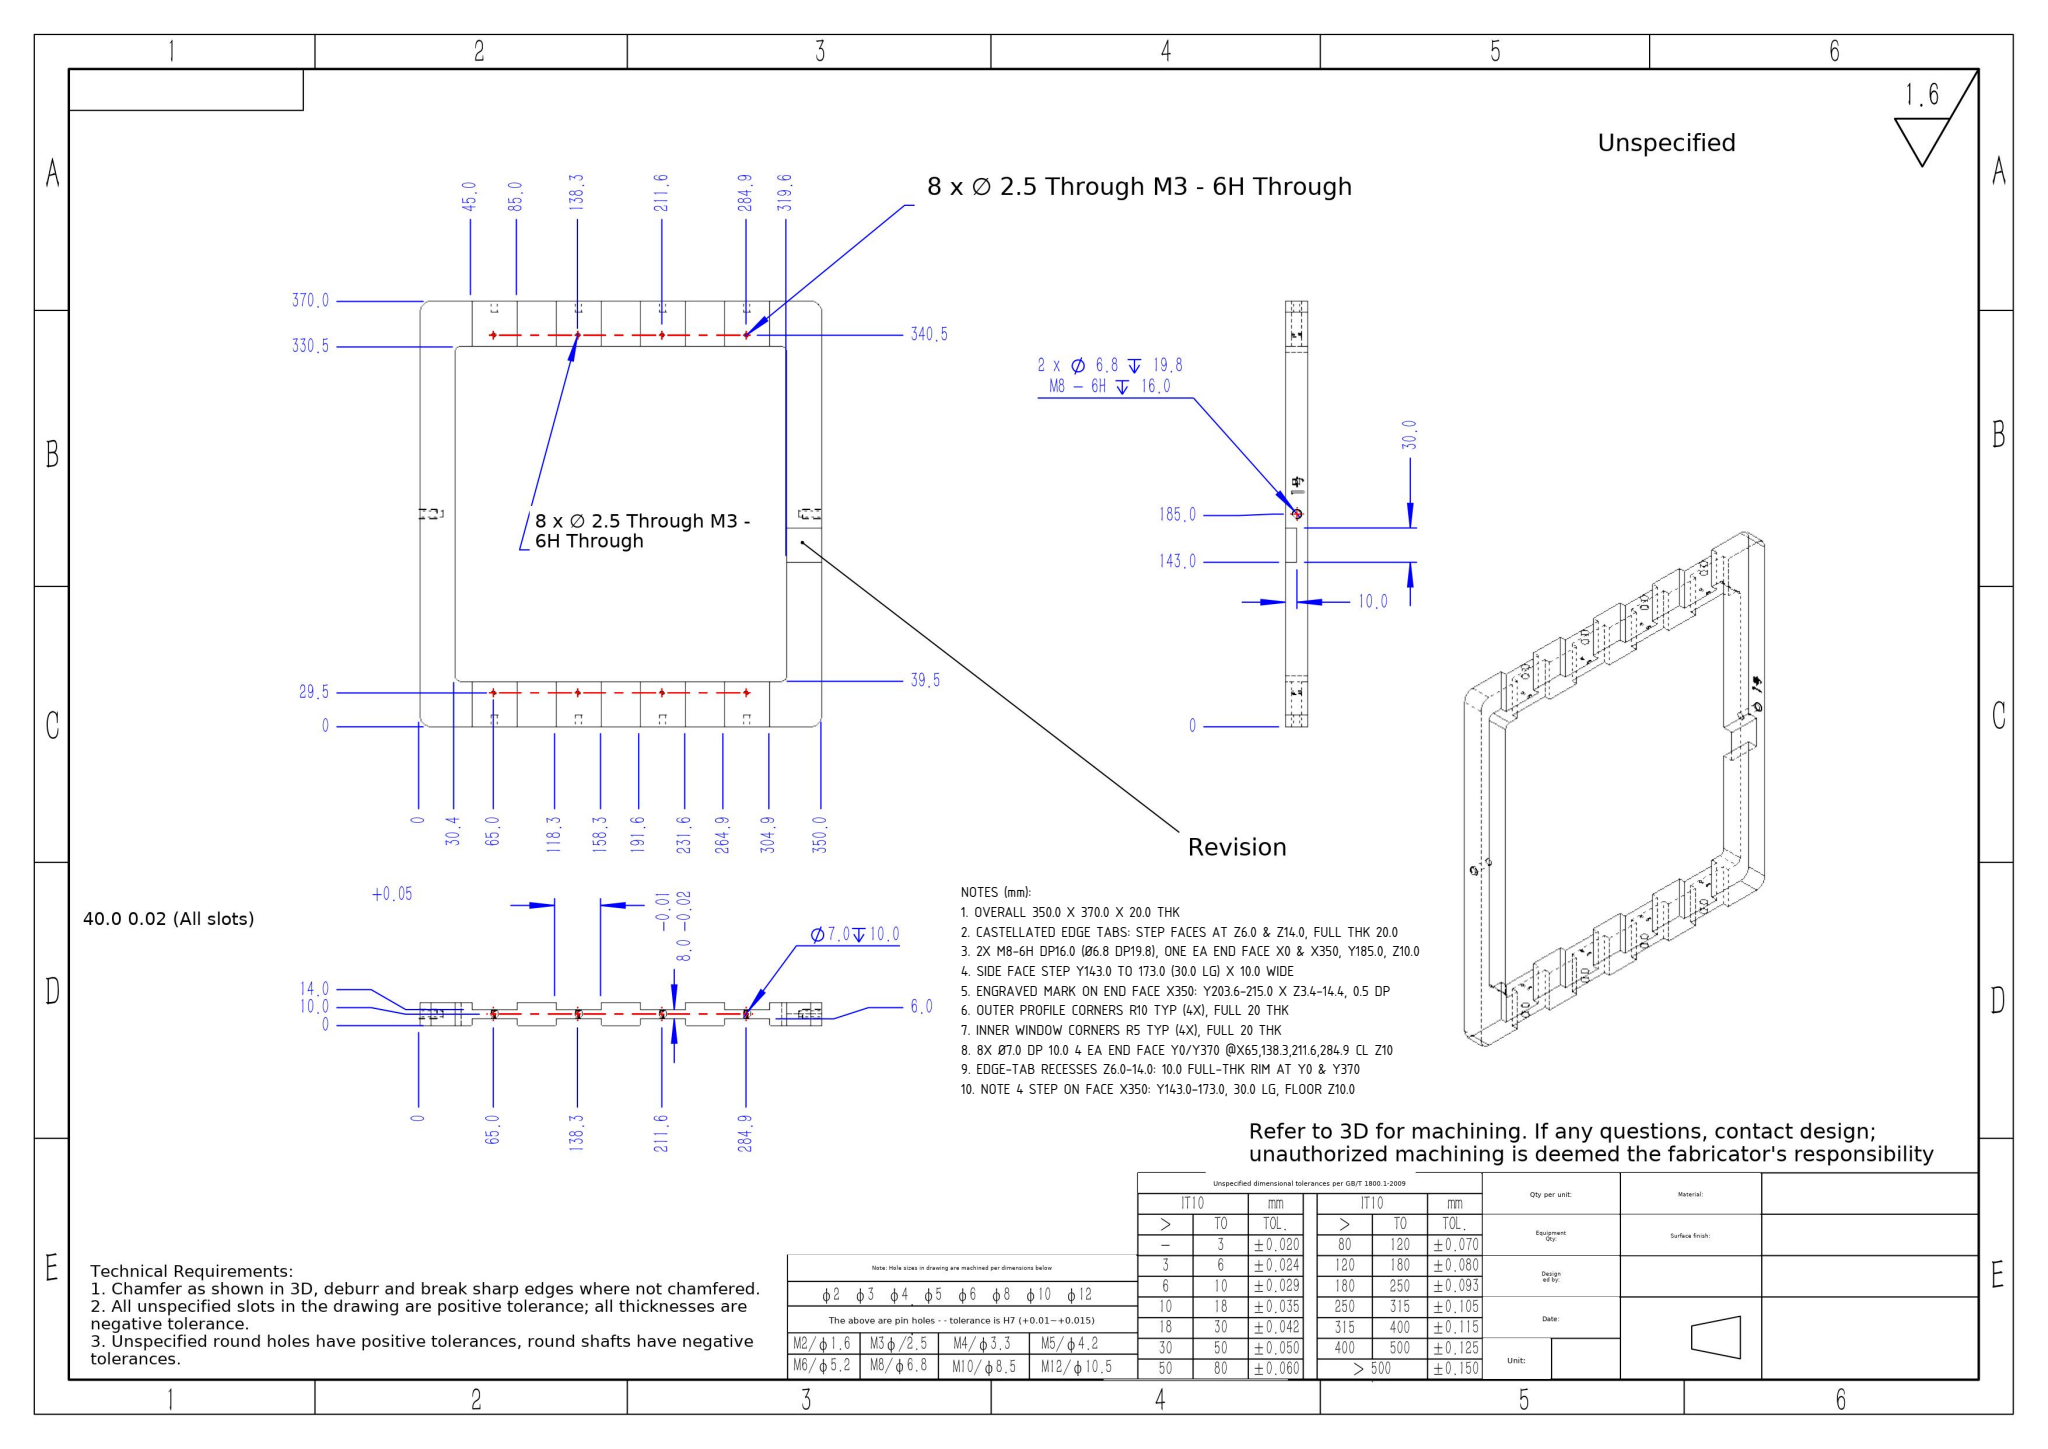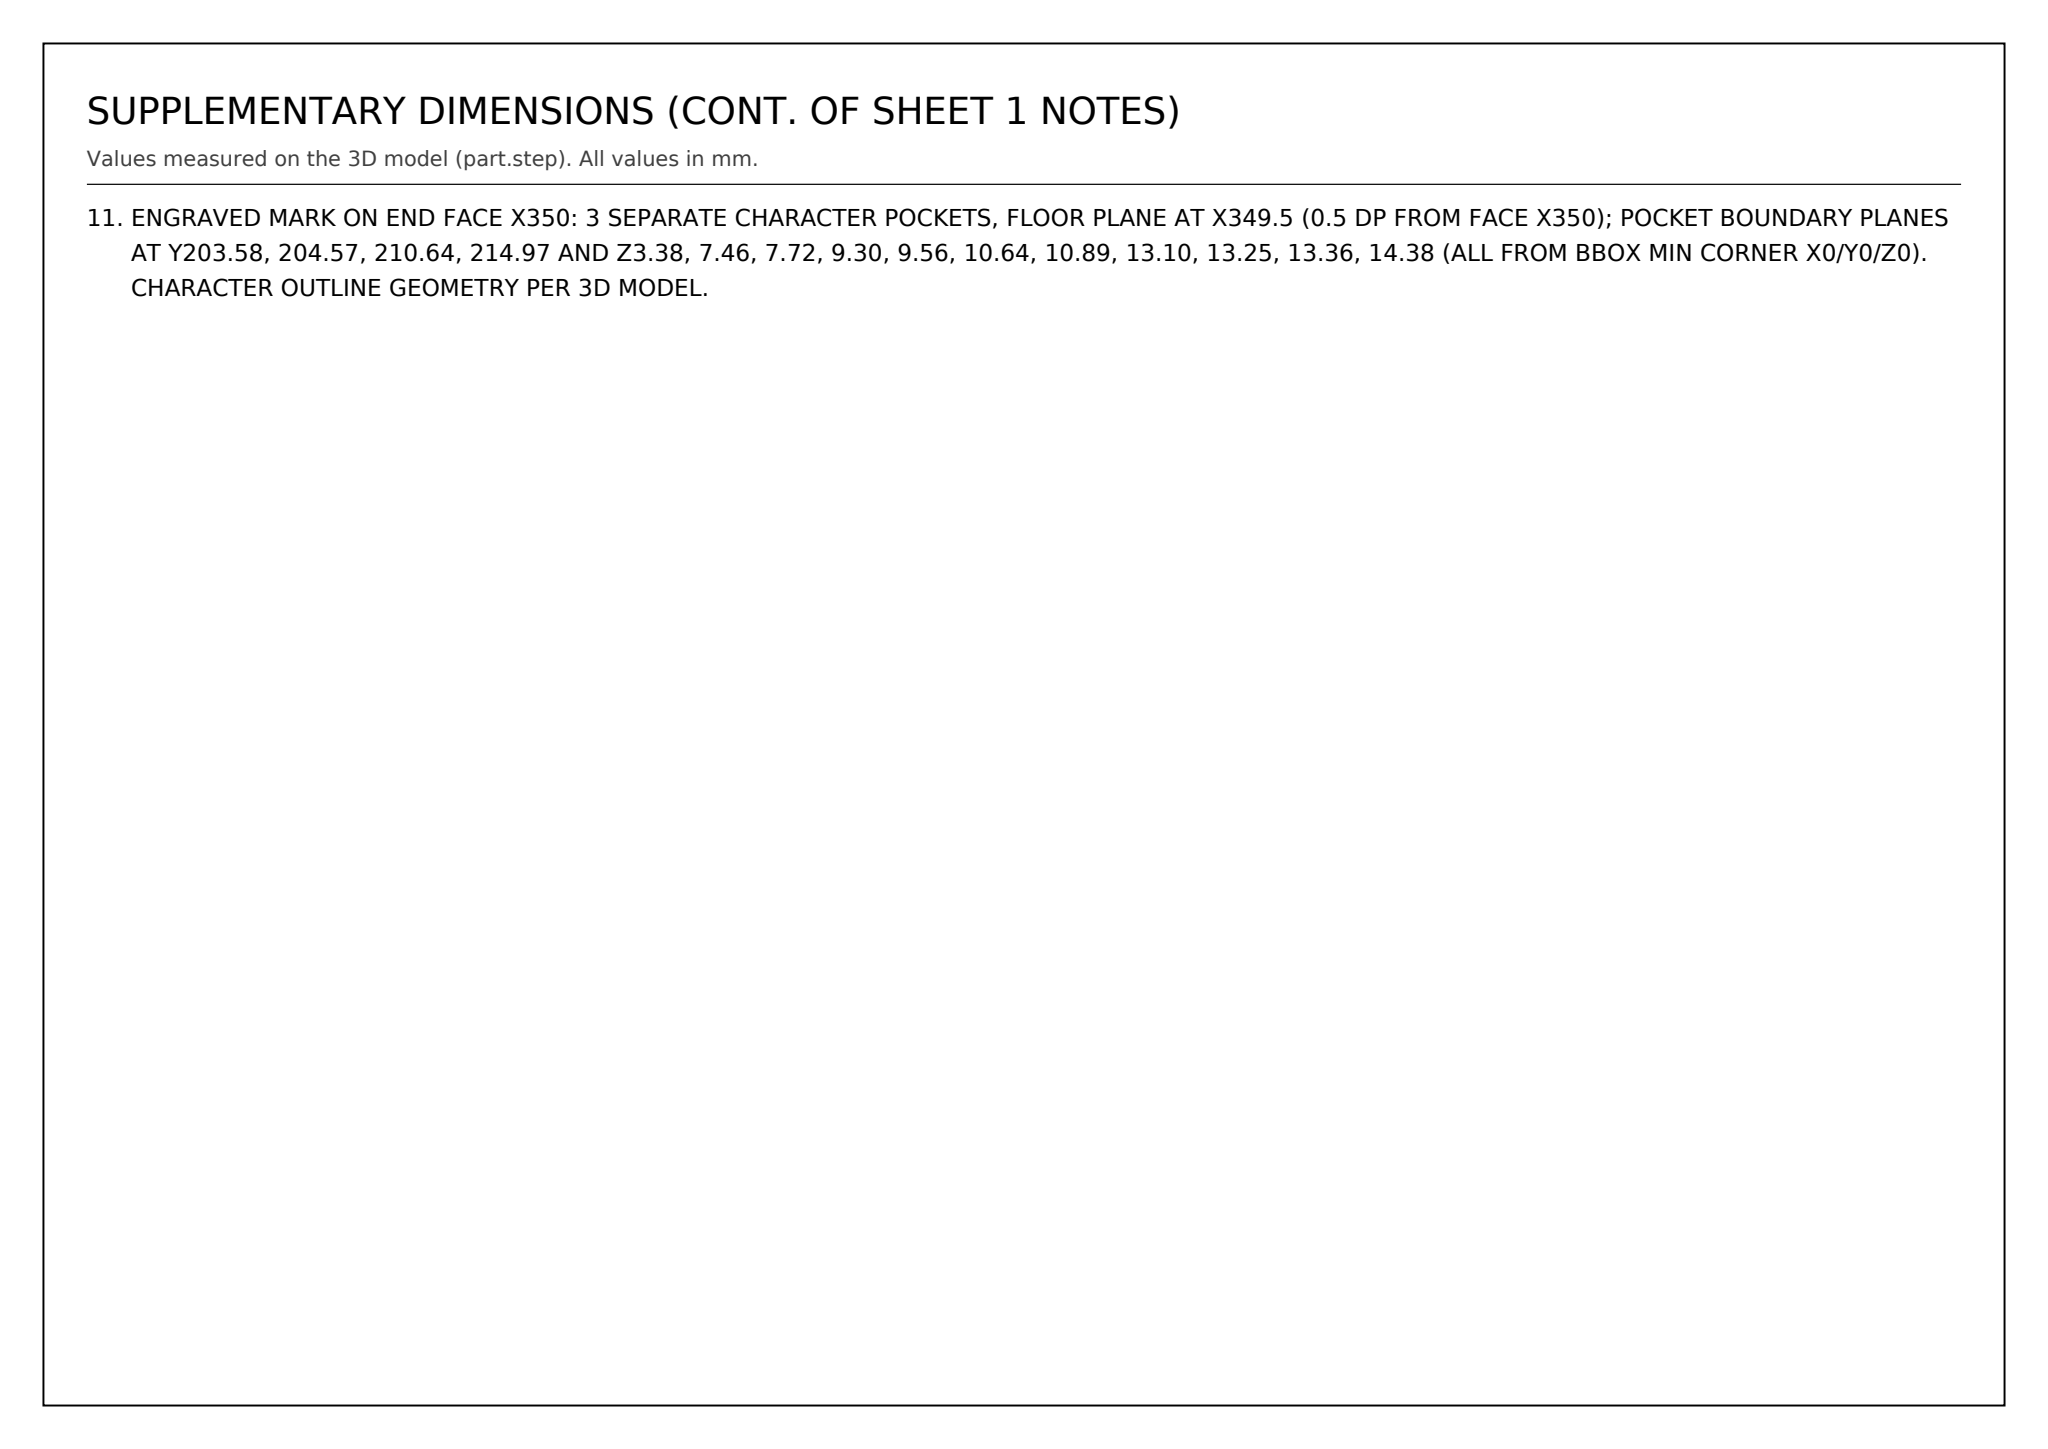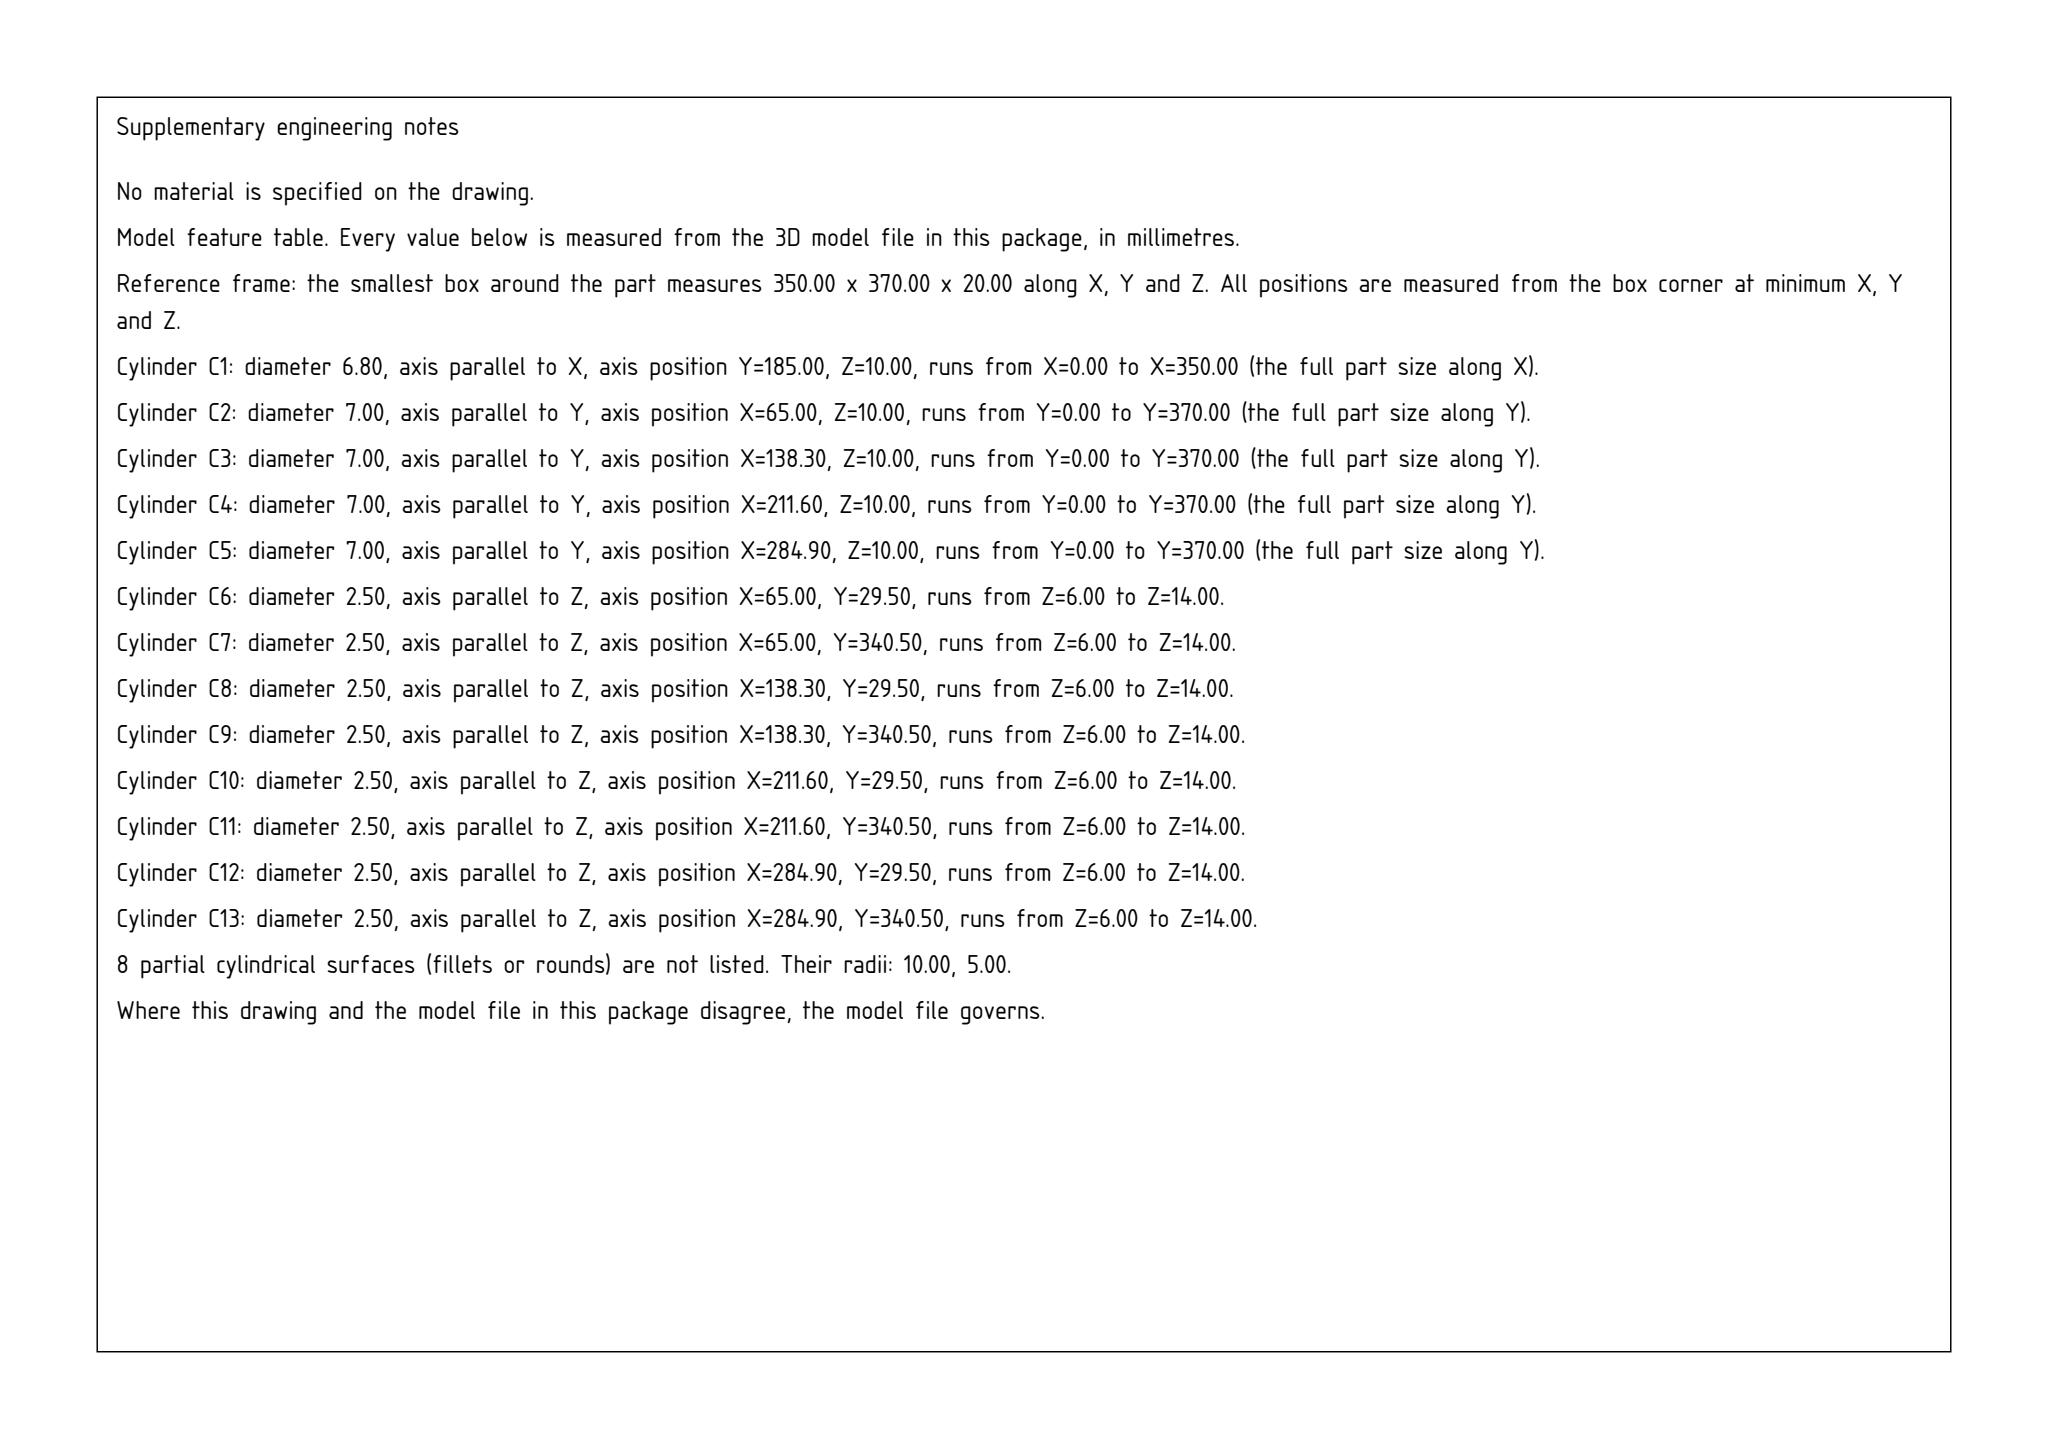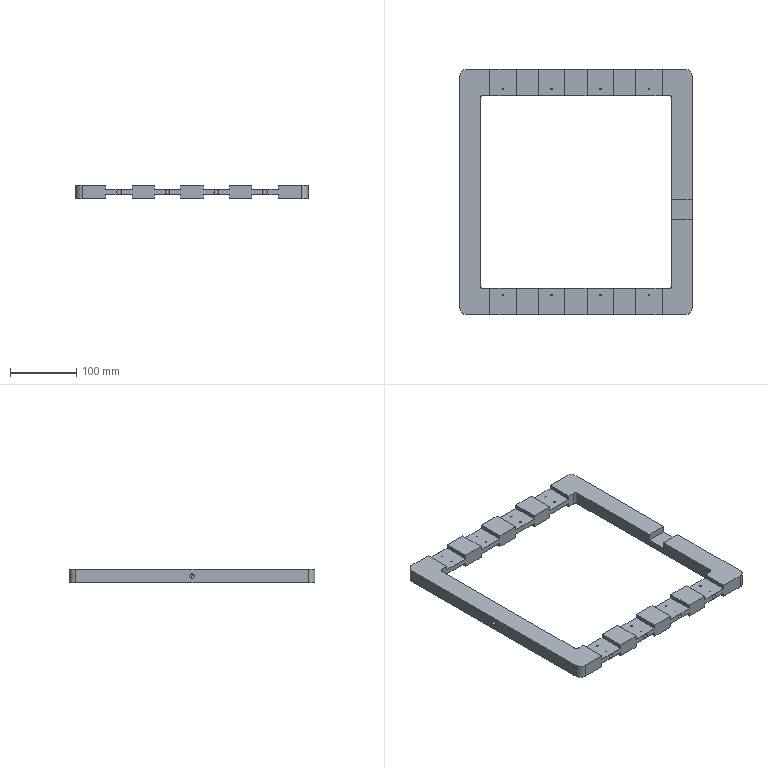Part | SolidWorks | mm | 1 solid | 179 faces | box 350 x 370 x 20 mm | volume 739874 mm3 | plane 124 | cylinder 44 | spline 7 | cone 4 | commonest cylinder face diameters 2.5 x16 7 x16 6.8 x4 20 x4 10 x4
Drawing notes:
OVERALL 350.0 X 370.0 X 20.0 THK | from the solid: bbox_xyz 350.0 x 370.0 x 20.0
CASTELLATED EDGE TABS: STEP FACES AT Z6.0 & Z14.0, FULL THK 20.0 | from the solid: z planes 0, 6.0, 14.0, 20.0, 8 faces each on tab edges
2X M8-6H DP16.0 (Ø6.8 DP19.8), ONE EA END FACE X0 & X350, Y185.0, Z10.0 | from the solid: Ø6.8 axis x at [-,185.0,10.0] L19.8, both x=0 and x=350 faces
SIDE FACE STEP Y143.0 TO 173.0 (30.0 LG) X 10.0 WIDE | from the solid: y planes 143.0 & 173.0 (delta 30.0); 10.0 width dim in right view
ENGRAVED MARK ON END FACE X350: Y203.6-215.0 X Z3.4-14.4, 0.5 DP | from the solid: x planes 349.5 & 350.0 (0.5 deep); y 203.58-214.97; z 3.38-14.38
OUTER PROFILE CORNERS R10 TYP (4X), FULL 20 THK | from the solid: Ø20 z-axis cylinders at (10,10),(10,360),(340,10),(340,360), len 20 = R10 at the 4 bbox corners of 350x370x20
INNER WINDOW CORNERS R5 TYP (4X), FULL 20 THK | from the solid: Ø10 z-axis cylinders at (35.4,44.5),(35.4,325.5),(314.6,44.5),(314.6,325.5), len 20 = R5 at pocket corners
8X Ø7.0 DP 10.0 4 EA END FACE Y0/Y370 @X65,138.3,211.6,284.9 CL Z10 | from the solid: Ø7.0 y-axis holes, depth 10, at X=65/138.3/211.6/284.9, Z=10, one from each of Y0 and Y370 faces (8 total)
EDGE-TAB RECESSES Z6.0-14.0: 10.0 FULL-THK RIM AT Y0 & Y370 | from the solid: y-planes 10.0 (x4) and 360.0 (x4) bound recess regions between z=6.0 and z=14.0; outer faces y=0.0 and y=370.0, bbox Y370.0
NOTE 4 STEP ON FACE X350: Y143.0-173.0, 30.0 LG, FLOOR Z10.0 | from the solid: y-planes 143.0 & 173.0 (30.0 apart), single z-plane 10.0 = step floor; x=350.0 face occurs 2x (split by step) vs x=0.0 face 1x
ENGRAVED MARK ON END FACE X350: 3 SEPARATE CHARACTER POCKETS, FLOOR PLANE AT X349.5 (0.5 DP FROM FACE X350); POCKET BOUNDARY PLANES AT Y203.58, 204.57, 210.64, 214.97 AND Z3.38, 7.46, 7.72, 9.30, 9.56, 10.64, 10.89, 13.10, 13.25, 13.36, 14.38 (ALL FROM BBOX MIN CORNER X0/Y0/Z0). CHARACTER OUTLINE GEOMETRY PER 3D MODEL. | from the solid: axis_planes[x,349.5]:3 (engraved floor, 0.5 below x=350 face); axis_planes y=203.58, 204.57, 210.64, 214.97; axis_planes z=3.38, 7.46, 7.72, 9.30, 9.56, 10.64, 10.89, 13.10, 13.25, 13.36, 14.38
build123d program:
from build123d import *

# Parameters (mm, degrees)
SKETCH1_W                 = 350
SKETCH1_H                 = 370
BOSS_EXTRUDE1_DEPTH       = 10
FILLET1_R                 = 10
SKETCH2_W                 = 289.2
SKETCH2_H                 = 291
CUT_EXTRUDE1_DEPTH        = 174
CUT_EXTRUDE2_DEPTH        = 0.5
SKETCH4_W                 = 2.202
SKETCH4_H                 = 4.327
CUT_EXTRUDE3_DEPTH        = 0.5
SKETCH5_W                 = 40
SKETCH5_H                 = 6
CUT_EXTRUDE4_DEPTH        = 410.42
SKETCH6_R                 = 3.5
CUT_EXTRUDE5_DEPTH        = 10
M3_TAPPED_HOLE1_D         = 2.5
LPATTERN1_COUNT           = 4
LPATTERN1_PITCH           = 73.3
LPATTERN1_COPY_1_SKETCH_W = 40
LPATTERN1_COPY_1_SKETCH_H = 6
LPATTERN1_COPY_1_DEPTH    = 410.42
LPATTERN1_COPY_2_SKETCH_W = 40
LPATTERN1_COPY_2_SKETCH_H = 6
LPATTERN1_COPY_2_DEPTH    = 410.42
LPATTERN1_COPY_3_SKETCH_W = 40
LPATTERN1_COPY_3_SKETCH_H = 6
LPATTERN1_COPY_3_DEPTH    = 410.42
LPATTERN1_COPY_4_SKETCH_R = 3.5
LPATTERN1_COPY_4_DEPTH    = 10
LPATTERN1_COPY_5_SKETCH_R = 3.5
LPATTERN1_COPY_5_DEPTH    = 10
LPATTERN1_COPY_6_SKETCH_R = 3.5
LPATTERN1_COPY_6_DEPTH    = 10
LPATTERN1_COPY_7_D        = 2.5
LPATTERN1_COPY_8_D        = 2.5
LPATTERN1_COPY_9_D        = 2.5
FILLET2_R                 = 5
SKETCH11_W                = 30.4
SKETCH11_H                = 30
CUT_EXTRUDE6_DEPTH        = 10


with BuildPart() as part:
    # Sketch1 → Boss-Extrude1 (new, symmetric)
    with BuildSketch(Plane.XY):
        Rectangle(SKETCH1_W, SKETCH1_H)
    extrude(amount=BOSS_EXTRUDE1_DEPTH, both=True)

    # Fillet1
    fillet1_edges = [part.edges().sort_by_distance(p)[0] for p in [
        (-175, 185, 0),
        (175, 185, 0),
        (175, -185, 0),
        (-175, -185, 0),
    ]]
    fillet(fillet1_edges, radius=FILLET1_R)

    # Sketch2 → Cut-Extrude1 (cut)
    with BuildSketch(Plane.XY.offset(10)):
        Rectangle(SKETCH2_W, SKETCH2_H)
    extrude(amount=-CUT_EXTRUDE1_DEPTH, mode=Mode.SUBTRACT)

    # Sketch3 → Cut-Extrude2 (cut)
    with BuildSketch(Plane(origin=(175, 0, 0), x_dir=(0, 0, -1), z_dir=(1, 0, 0))):
        Polygon((-4.375, 17.532), (-4.375, 19.566), (6.625, 19.566), (6.625, 18.579), (-3.247, 18.579), (-3.247, 16.887), align=None)
    extrude(amount=-CUT_EXTRUDE2_DEPTH, mode=Mode.SUBTRACT)

    # Sketch4 → Cut-Extrude3 (cut)
    # profile 1 of 2: a face of its own
    with BuildSketch(Plane(origin=(175, 0, 0), x_dir=(0, 0, -1), z_dir=(1, 0, 0))):
        with BuildLine():
            add(Edge.make_bspline(
                [(-2.988, 30.571), (-2.832, 30.571), (-2.534, 30.57), (-2.11, 30.575), (-1.728, 30.577), (-1.391, 30.582), (-1.097, 30.589), (-0.8468, 30.594), (-0.6401, 30.604), (-0.5168, 30.611), (-0.4623, 30.615)],
                knots=[0, 0, 0, 0, 1.482, 2.827, 4.034, 5.105, 6.034, 6.826, 7.481, 8, 8, 8, 8], degree=3))
            Line((-0.4623, 30.615), (-0.2027, 29.966))
            Line((-0.2027, 29.966), (-0.6354, 29.966))
            Line((-0.6354, 29.966), (-0.6354, 25.639))
            Line((-0.6354, 25.639), (-0.2459, 25.639))
            Line((-0.2459, 25.639), (-0.02959, 24.99))
            add(Edge.make_bspline(
                [(-0.02959, 24.99), (-0.1759, 24.997), (-0.4734, 25.011), (-0.9264, 25.023), (-1.393, 25.031), (-1.868, 25.034), (-2.342, 25.031), (-2.807, 25.023), (-3.259, 25.011), (-3.556, 24.997), (-3.703, 24.99)],
                knots=[0, 0, 0, 0, 0.9569, 1.945, 2.96, 4.003, 5.047, 6.059, 7.043, 8, 8, 8, 8], degree=3))
            Line((-3.703, 24.99), (-3.357, 25.639))
            Line((-3.357, 25.639), (-3.357, 29.922))
            Line((-3.357, 29.922), (-3.815, 30.312))
            Line((-3.815, 30.312), (-3.292, 30.918))
            Line((-3.292, 30.918), (-2.988, 30.571))
        make_face()
        with Locations((-1.996, 27.802)):
            Rectangle(SKETCH4_W, SKETCH4_H, mode=Mode.SUBTRACT)
    # profile 2 of 2: a face of its own
    with BuildSketch(Plane(origin=(175, 0, 0), x_dir=(0, 0, -1), z_dir=(1, 0, 0))):
        with BuildLine():
            add(Edge.make_bspline(
                [(2.756, 30.831), (2.846, 30.815), (3.021, 30.785), (3.277, 30.736), (3.518, 30.69), (3.745, 30.643), (3.956, 30.597), (4.153, 30.552), (4.336, 30.509), (4.504, 30.466), (4.657, 30.423), (4.795, 30.379), (4.918, 30.338), (5.027, 30.298), (5.122, 30.259), (5.201, 30.218), (5.268, 30.181), (5.361, 30.106), (5.477, 29.993), (5.613, 29.842), (5.726, 29.691), (5.817, 29.529), (5.897, 29.344), (5.974, 29.118), (6.055, 28.845), (6.106, 28.645), (6.134, 28.538)],
                knots=[0, 0, 0, 0, 1.466, 2.848, 4.161, 5.391, 6.545, 7.622, 8.623, 9.549, 10.392, 11.162, 11.856, 12.475, 13.022, 13.492, 13.898, 14.233, 15.399, 16.488, 17.484, 18.417, 19.442, 20.709, 22.225, 24, 24, 24, 24], degree=3))
            add(Edge.make_bspline(
                [(6.134, 28.538), (6.08, 28.527), (5.97, 28.504), (5.814, 28.422), (5.662, 28.308), (5.516, 28.156), (5.373, 27.969), (5.237, 27.744), (5.102, 27.484), (5.022, 27.295), (4.98, 27.196)],
                knots=[0, 0, 0, 0, 0.7104, 1.457, 2.272, 3.178, 4.195, 5.332, 6.601, 8, 8, 8, 8], degree=3))
            Line((4.98, 27.196), (4.809, 27.24))
            add(Edge.make_bspline(
                [(4.809, 27.24), (4.835, 27.334), (4.888, 27.515), (4.959, 27.779), (5.015, 28.025), (5.067, 28.25), (5.103, 28.457), (5.131, 28.645), (5.149, 28.814), (5.151, 28.92), (5.151, 28.97)],
                knots=[0, 0, 0, 0, 1.326, 2.563, 3.702, 4.748, 5.698, 6.554, 7.319, 8, 8, 8, 8], degree=3))
            add(Edge.make_bspline(
                [(5.151, 28.97), (5.15, 29.009), (5.146, 29.091), (5.12, 29.22), (5.077, 29.361), (5.043, 29.476), (4.999, 29.556), (4.953, 29.596), (4.894, 29.638), (4.815, 29.677), (4.722, 29.719), (4.61, 29.76), (4.481, 29.802), (4.334, 29.843), (4.17, 29.884), (3.989, 29.928), (3.79, 29.968), (3.575, 30.013), (3.342, 30.053), (3.091, 30.097), (2.824, 30.14), (2.639, 30.168), (2.544, 30.182)],
                knots=[0, 0, 0, 0, 0.7317, 1.557, 2.484, 3.53, 3.825, 4.205, 4.664, 5.213, 5.857, 6.614, 7.467, 8.436, 9.503, 10.681, 11.965, 13.351, 14.855, 16.46, 18.175, 20, 20, 20, 20], degree=3))
            Line((2.544, 30.182), (2.544, 26.201))
            Line((2.544, 26.201), (2.89, 25.812))
            Line((2.89, 25.812), (2.28, 25.293))
            add(Edge.make_bspline(
                [(2.28, 25.293), (2.248, 25.342), (2.182, 25.443), (2.051, 25.575), (1.891, 25.692), (1.704, 25.795), (1.491, 25.89), (1.252, 25.986), (0.984, 26.074), (0.7959, 26.129), (0.698, 26.158)],
                knots=[0, 0, 0, 0, 0.7634, 1.56, 2.409, 3.327, 4.334, 5.448, 6.672, 8, 8, 8, 8], degree=3))
            Line((0.698, 26.158), (0.698, 23.692))
            Line((0.698, 23.692), (0.7845, 23.302))
            Line((0.7845, 23.302), (0.4384, 22.956))
            Line((0.4384, 22.956), (0.4384, 31.307))
            Line((0.4384, 31.307), (-0.1241, 31.87))
            Line((-0.1241, 31.87), (0.698, 32.648))
            Line((0.698, 32.648), (0.698, 26.894))
            Line((0.698, 26.894), (2.285, 26.288))
            Line((2.285, 26.288), (2.285, 30.139))
            Line((2.285, 30.139), (1.809, 30.615))
            Line((1.809, 30.615), (2.456, 31.264))
            Line((2.456, 31.264), (2.756, 30.831))
        make_face()
    extrude(amount=-CUT_EXTRUDE3_DEPTH, mode=Mode.SUBTRACT)

    # Sketch5 → Cut-Extrude4 (cut, through all)
    with BuildSketch(Plane(origin=(0, 185, 0), x_dir=(1, 0, 0), z_dir=(0, 1, 0))):
        with Locations((109.9, -7)):
            Rectangle(SKETCH5_W, SKETCH5_H)
    cut_extrude4 = extrude(amount=-CUT_EXTRUDE4_DEPTH, mode=Mode.SUBTRACT)

    # Mirror1: Cut-Extrude4 across plane
    add(cut_extrude4.mirror(Plane.XY), mode=Mode.SUBTRACT)

    # Sketch6 → Cut-Extrude5 (cut)
    with BuildSketch(Plane(origin=(0, 185, 0), x_dir=(1, 0, 0), z_dir=(0, 1, 0))):
        with Locations(Location((109.9, 0, 0), (0, 0, 180))):
            Circle(SKETCH6_R)
    cut_extrude5 = extrude(amount=-CUT_EXTRUDE5_DEPTH, mode=Mode.SUBTRACT)

    # M3 Tapped Hole1 (through all)
    with Locations(Plane(origin=(0, 0, -10), x_dir=(-1, 0, 0), z_dir=(0, 0, -1))):
        with Locations((-109.9, 155.5)):
            m3_tapped_hole1 = Hole(M3_TAPPED_HOLE1_D / 2)

    # Mirror2: Cut-Extrude5, M3 Tapped Hole1 across plane
    add(cut_extrude5.mirror(Plane.ZX), mode=Mode.SUBTRACT)
    add(m3_tapped_hole1.mirror(Plane.ZX), mode=Mode.SUBTRACT)

    # LPattern1: Cut-Extrude4, Cut-Extrude5, M3 Tapped Hole1 ×4
    with Locations(*[(-i * LPATTERN1_PITCH, 0, 0) for i in range(1, LPATTERN1_COUNT)]):
        add(cut_extrude4, mode=Mode.SUBTRACT)
        add(cut_extrude5, mode=Mode.SUBTRACT)
        add(m3_tapped_hole1, mode=Mode.SUBTRACT)

    # LPattern1 copy 1 sketch → LPattern1 copy 1 (cut, through all)
    with BuildSketch(Plane(origin=(-73.3, 185, 0), x_dir=(1, 0, 0), z_dir=(0, 1, 0))):
        with Locations((109.9, 7)):
            Rectangle(LPATTERN1_COPY_1_SKETCH_W, LPATTERN1_COPY_1_SKETCH_H)
    extrude(amount=-LPATTERN1_COPY_1_DEPTH, mode=Mode.SUBTRACT)

    # LPattern1 copy 2 sketch → LPattern1 copy 2 (cut, through all)
    with BuildSketch(Plane(origin=(-146.6, 185, 0), x_dir=(1, 0, 0), z_dir=(0, 1, 0))):
        with Locations((109.9, 7)):
            Rectangle(LPATTERN1_COPY_2_SKETCH_W, LPATTERN1_COPY_2_SKETCH_H)
    extrude(amount=-LPATTERN1_COPY_2_DEPTH, mode=Mode.SUBTRACT)

    # LPattern1 copy 3 sketch → LPattern1 copy 3 (cut, through all)
    with BuildSketch(Plane(origin=(-219.9, 185, 0), x_dir=(1, 0, 0), z_dir=(0, 1, 0))):
        with Locations((109.9, 7)):
            Rectangle(LPATTERN1_COPY_3_SKETCH_W, LPATTERN1_COPY_3_SKETCH_H)
    extrude(amount=-LPATTERN1_COPY_3_DEPTH, mode=Mode.SUBTRACT)

    # LPattern1 copy 4 sketch → LPattern1 copy 4 (cut)
    with BuildSketch(Plane(origin=(-73.3, -185, 0), x_dir=(1, 0, 0), z_dir=(0, -1, 0))):
        with Locations((109.9, 0)):
            Circle(LPATTERN1_COPY_4_SKETCH_R)
    extrude(amount=-LPATTERN1_COPY_4_DEPTH, mode=Mode.SUBTRACT)

    # LPattern1 copy 5 sketch → LPattern1 copy 5 (cut)
    with BuildSketch(Plane(origin=(-146.6, -185, 0), x_dir=(1, 0, 0), z_dir=(0, -1, 0))):
        with Locations((109.9, 0)):
            Circle(LPATTERN1_COPY_5_SKETCH_R)
    extrude(amount=-LPATTERN1_COPY_5_DEPTH, mode=Mode.SUBTRACT)

    # LPattern1 copy 6 sketch → LPattern1 copy 6 (cut)
    with BuildSketch(Plane(origin=(-219.9, -185, 0), x_dir=(1, 0, 0), z_dir=(0, -1, 0))):
        with Locations((109.9, 0)):
            Circle(LPATTERN1_COPY_6_SKETCH_R)
    extrude(amount=-LPATTERN1_COPY_6_DEPTH, mode=Mode.SUBTRACT)

    # LPattern1 copy 7 (through all)
    with Locations(Plane(origin=(-73.3, 0, -10), x_dir=(-1, 0, 0), z_dir=(0, 0, -1))):
        with Locations((-109.9, -155.5)):
            Hole(LPATTERN1_COPY_7_D / 2)

    # LPattern1 copy 8 (through all)
    with Locations(Plane(origin=(-146.6, 0, -10), x_dir=(-1, 0, 0), z_dir=(0, 0, -1))):
        with Locations((-109.9, -155.5)):
            Hole(LPATTERN1_COPY_8_D / 2)

    # LPattern1 copy 9 (through all)
    with Locations(Plane(origin=(-219.9, 0, -10), x_dir=(-1, 0, 0), z_dir=(0, 0, -1))):
        with Locations((-109.9, -155.5)):
            Hole(LPATTERN1_COPY_9_D / 2)

    # Sketch10 → M8 Tapped Hole1 (revolve, cut)
    with BuildSketch(Plane(origin=(175, 0, 0), x_dir=(0, 0, -1), z_dir=(0, 1, 0))):
        Polygon((0, 0), (0, 21.843), (3.4, 19.8), (3.4, 0), align=None)
    m8_tapped_hole1 = revolve(axis=Axis((181.35, 0, 0), (-1, 0, 0)), mode=Mode.SUBTRACT)

    # Mirror3: M8 Tapped Hole1 across plane
    add(m8_tapped_hole1.mirror(Plane(origin=(0, 0, 0), x_dir=(0, 0, 1), z_dir=(1, 0, 0))), mode=Mode.SUBTRACT)

    # Fillet2
    fillet2_edges = [part.edges().sort_by_distance(p)[0] for p in [
        (-144.6, -145.5, 0),
        (-144.6, 145.5, 0),
        (144.6, 145.5, 0),
        (144.6, -145.5, 0),
    ]]
    fillet(fillet2_edges, radius=FILLET2_R)

    # Sketch11 → Cut-Extrude6 (cut)
    with BuildSketch(Plane.XY.offset(10)):
        with Locations((159.8, -27)):
            Rectangle(SKETCH11_W, SKETCH11_H)
    extrude(amount=-CUT_EXTRUDE6_DEPTH, mode=Mode.SUBTRACT)


solid = part.part